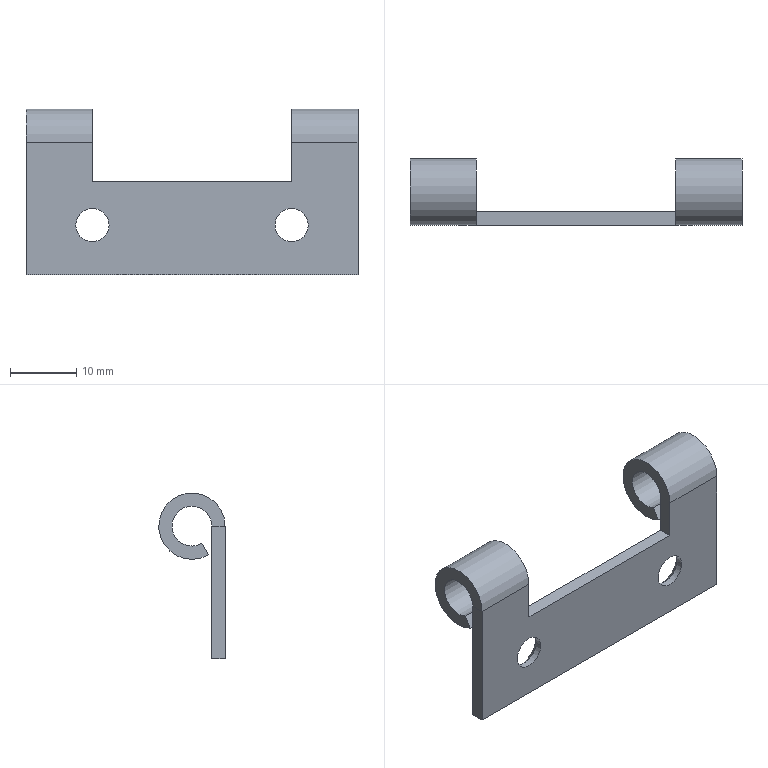Component | SolidWorks | Hinge-1_Hinge1-1 | 1 solid | 24 faces | box 50 x 10 x 25 mm | volume 2381 mm3 | plane 12 | cylinder 8 | cone 4 | commonest cylinder face diameters 5 x4 6 x2 10 x2
STEP:
#1=CARTESIAN_POINT('',(47.547,58.634,57.439));
#2=VERTEX_POINT('',#1);
#3=CARTESIAN_POINT('',(47.35,58.634,57.439));
#4=VERTEX_POINT('',#3);
#5=CARTESIAN_POINT('',(47.448,58.634,57.439));
#6=DIRECTION('',(0.,1.,0.));
#7=DIRECTION('',(-1.,0.,0.));
#8=AXIS2_PLACEMENT_3D('',#5,#6,#7);
#9=CIRCLE('',#8,0.09843);
#10=EDGE_CURVE('',#2,#4,#9,.T.);
#11=ORIENTED_EDGE('',*,*,#10,.F.);
#12=CARTESIAN_POINT('',(47.586,58.674,57.439));
#13=VERTEX_POINT('',#12);
#14=CARTESIAN_POINT('',(47.586,58.674,57.439));
#15=DIRECTION('',(0.7071,0.7071,0.));
#16=VECTOR('',#15,39.37);
#17=LINE('',#14,#16);
#18=EDGE_CURVE('',#2,#13,#17,.T.);
#19=ORIENTED_EDGE('',*,*,#18,.T.);
#20=CARTESIAN_POINT('',(47.31,58.674,57.439));
#21=VERTEX_POINT('',#20);
#22=CARTESIAN_POINT('',(47.448,58.674,57.439));
#23=DIRECTION('',(0.,-1.,-0.));
#24=DIRECTION('',(-1.,0.,0.));
#25=AXIS2_PLACEMENT_3D('',#22,#23,#24);
#26=CIRCLE('',#25,0.1378);
#27=EDGE_CURVE('',#21,#13,#26,.T.);
#28=ORIENTED_EDGE('',*,*,#27,.F.);
#29=CARTESIAN_POINT('',(47.31,58.674,57.439));
#30=DIRECTION('',(-0.7071,0.7071,0.));
#31=VECTOR('',#30,39.37);
#32=LINE('',#29,#31);
#33=EDGE_CURVE('',#4,#21,#32,.T.);
#34=ORIENTED_EDGE('',*,*,#33,.F.);
#35=EDGE_LOOP('',(#11,#19,#28,#34));
#36=FACE_OUTER_BOUND('',#35,.T.);
#37=CARTESIAN_POINT('',(47.448,58.674,57.439));
#38=DIRECTION('',(0.,1.,0.));
#39=DIRECTION('',(-1.,0.,0.));
#40=AXIS2_PLACEMENT_3D('',#37,#38,#39);
#41=CONICAL_SURFACE('',#40,0.1378,0.7854);
#42=ADVANCED_FACE('',(#36),#41,.F.);
#43=CARTESIAN_POINT('',(46.366,58.634,57.439));
#44=VERTEX_POINT('',#43);
#45=CARTESIAN_POINT('',(46.169,58.634,57.439));
#46=VERTEX_POINT('',#45);
#47=CARTESIAN_POINT('',(46.267,58.634,57.439));
#48=DIRECTION('',(0.,1.,0.));
#49=DIRECTION('',(-1.,0.,0.));
#50=AXIS2_PLACEMENT_3D('',#47,#48,#49);
#51=CIRCLE('',#50,0.09843);
#52=EDGE_CURVE('',#44,#46,#51,.T.);
#53=ORIENTED_EDGE('',*,*,#52,.F.);
#54=CARTESIAN_POINT('',(46.405,58.674,57.439));
#55=VERTEX_POINT('',#54);
#56=CARTESIAN_POINT('',(46.405,58.674,57.439));
#57=DIRECTION('',(0.7071,0.7071,0.));
#58=VECTOR('',#57,39.37);
#59=LINE('',#56,#58);
#60=EDGE_CURVE('',#44,#55,#59,.T.);
#61=ORIENTED_EDGE('',*,*,#60,.T.);
#62=CARTESIAN_POINT('',(46.129,58.674,57.439));
#63=VERTEX_POINT('',#62);
#64=CARTESIAN_POINT('',(46.267,58.674,57.439));
#65=DIRECTION('',(0.,-1.,-0.));
#66=DIRECTION('',(-1.,0.,0.));
#67=AXIS2_PLACEMENT_3D('',#64,#65,#66);
#68=CIRCLE('',#67,0.1378);
#69=EDGE_CURVE('',#63,#55,#68,.T.);
#70=ORIENTED_EDGE('',*,*,#69,.F.);
#71=CARTESIAN_POINT('',(46.129,58.674,57.439));
#72=DIRECTION('',(-0.7071,0.7071,0.));
#73=VECTOR('',#72,39.37);
#74=LINE('',#71,#73);
#75=EDGE_CURVE('',#46,#63,#74,.T.);
#76=ORIENTED_EDGE('',*,*,#75,.F.);
#77=EDGE_LOOP('',(#53,#61,#70,#76));
#78=FACE_OUTER_BOUND('',#77,.T.);
#79=CARTESIAN_POINT('',(46.267,58.674,57.439));
#80=DIRECTION('',(0.,1.,0.));
#81=DIRECTION('',(-1.,0.,0.));
#82=AXIS2_PLACEMENT_3D('',#79,#80,#81);
#83=CONICAL_SURFACE('',#82,0.1378,0.7854);
#84=ADVANCED_FACE('',(#78),#83,.F.);
#85=ORIENTED_EDGE('',*,*,#52,.T.);
#86=CARTESIAN_POINT('',(46.169,58.595,57.439));
#87=VERTEX_POINT('',#86);
#88=CARTESIAN_POINT('',(46.169,58.989,57.439));
#89=DIRECTION('',(0.,-1.,-0.));
#90=VECTOR('',#89,39.37);
#91=LINE('',#88,#90);
#92=EDGE_CURVE('',#46,#87,#91,.T.);
#93=ORIENTED_EDGE('',*,*,#92,.T.);
#94=CARTESIAN_POINT('',(46.366,58.595,57.439));
#95=VERTEX_POINT('',#94);
#96=CARTESIAN_POINT('',(46.267,58.595,57.439));
#97=DIRECTION('',(0.,-1.,-0.));
#98=DIRECTION('',(1.,0.,0.));
#99=AXIS2_PLACEMENT_3D('',#96,#97,#98);
#100=CIRCLE('',#99,0.09843);
#101=EDGE_CURVE('',#87,#95,#100,.T.);
#102=ORIENTED_EDGE('',*,*,#101,.T.);
#103=CARTESIAN_POINT('',(46.366,58.989,57.439));
#104=DIRECTION('',(0.,-1.,-0.));
#105=VECTOR('',#104,39.37);
#106=LINE('',#103,#105);
#107=EDGE_CURVE('',#44,#95,#106,.T.);
#108=ORIENTED_EDGE('',*,*,#107,.F.);
#109=EDGE_LOOP('',(#85,#93,#102,#108));
#110=FACE_OUTER_BOUND('',#109,.T.);
#111=CARTESIAN_POINT('',(46.267,58.989,57.439));
#112=DIRECTION('',(0.,-1.,-0.));
#113=DIRECTION('',(1.,0.,0.));
#114=AXIS2_PLACEMENT_3D('',#111,#112,#113);
#115=CYLINDRICAL_SURFACE('',#114,0.09843);
#116=ADVANCED_FACE('',(#110),#115,.F.);
#117=ORIENTED_EDGE('',*,*,#10,.T.);
#118=CARTESIAN_POINT('',(47.35,58.595,57.439));
#119=VERTEX_POINT('',#118);
#120=CARTESIAN_POINT('',(47.35,58.989,57.439));
#121=DIRECTION('',(0.,-1.,-0.));
#122=VECTOR('',#121,39.37);
#123=LINE('',#120,#122);
#124=EDGE_CURVE('',#4,#119,#123,.T.);
#125=ORIENTED_EDGE('',*,*,#124,.T.);
#126=CARTESIAN_POINT('',(47.547,58.595,57.439));
#127=VERTEX_POINT('',#126);
#128=CARTESIAN_POINT('',(47.448,58.595,57.439));
#129=DIRECTION('',(0.,-1.,-0.));
#130=DIRECTION('',(1.,0.,0.));
#131=AXIS2_PLACEMENT_3D('',#128,#129,#130);
#132=CIRCLE('',#131,0.09843);
#133=EDGE_CURVE('',#119,#127,#132,.T.);
#134=ORIENTED_EDGE('',*,*,#133,.T.);
#135=CARTESIAN_POINT('',(47.547,58.989,57.439));
#136=DIRECTION('',(0.,-1.,-0.));
#137=VECTOR('',#136,39.37);
#138=LINE('',#135,#137);
#139=EDGE_CURVE('',#2,#127,#138,.T.);
#140=ORIENTED_EDGE('',*,*,#139,.F.);
#141=EDGE_LOOP('',(#117,#125,#134,#140));
#142=FACE_OUTER_BOUND('',#141,.T.);
#143=CARTESIAN_POINT('',(47.448,58.989,57.439));
#144=DIRECTION('',(0.,-1.,-0.));
#145=DIRECTION('',(1.,0.,0.));
#146=AXIS2_PLACEMENT_3D('',#143,#144,#145);
#147=CYLINDRICAL_SURFACE('',#146,0.09843);
#148=ADVANCED_FACE('',(#142),#147,.F.);
#149=CARTESIAN_POINT('',(47.448,58.733,57.829));
#150=VERTEX_POINT('',#149);
#151=CARTESIAN_POINT('',(47.448,58.674,57.931));
#152=VERTEX_POINT('',#151);
#153=CARTESIAN_POINT('',(47.448,58.792,57.931));
#154=DIRECTION('',(1.,0.,0.));
#155=DIRECTION('',(0.,1.,0.));
#156=AXIS2_PLACEMENT_3D('',#153,#154,#155);
#157=CIRCLE('',#156,0.1181);
#158=EDGE_CURVE('',#150,#152,#157,.T.);
#159=ORIENTED_EDGE('',*,*,#158,.F.);
#160=CARTESIAN_POINT('',(47.842,58.733,57.829));
#161=VERTEX_POINT('',#160);
#162=CARTESIAN_POINT('',(47.842,58.733,57.829));
#163=DIRECTION('',(-1.,0.,0.));
#164=VECTOR('',#163,39.37);
#165=LINE('',#162,#164);
#166=EDGE_CURVE('',#161,#150,#165,.T.);
#167=ORIENTED_EDGE('',*,*,#166,.F.);
#168=CARTESIAN_POINT('',(47.842,58.674,57.931));
#169=VERTEX_POINT('',#168);
#170=CARTESIAN_POINT('',(47.842,58.792,57.931));
#171=DIRECTION('',(1.,0.,0.));
#172=DIRECTION('',(0.,1.,0.));
#173=AXIS2_PLACEMENT_3D('',#170,#171,#172);
#174=CIRCLE('',#173,0.1181);
#175=EDGE_CURVE('',#161,#169,#174,.T.);
#176=ORIENTED_EDGE('',*,*,#175,.T.);
#177=CARTESIAN_POINT('',(47.842,58.674,57.931));
#178=DIRECTION('',(-1.,0.,0.));
#179=VECTOR('',#178,39.37);
#180=LINE('',#177,#179);
#181=EDGE_CURVE('',#169,#152,#180,.T.);
#182=ORIENTED_EDGE('',*,*,#181,.T.);
#183=EDGE_LOOP('',(#159,#167,#176,#182));
#184=FACE_OUTER_BOUND('',#183,.T.);
#185=CARTESIAN_POINT('',(47.842,58.792,57.931));
#186=DIRECTION('',(-1.,0.,0.));
#187=DIRECTION('',(0.,-1.,0.));
#188=AXIS2_PLACEMENT_3D('',#185,#186,#187);
#189=CYLINDRICAL_SURFACE('',#188,0.1181);
#190=ADVANCED_FACE('',(#184),#189,.F.);
#191=CARTESIAN_POINT('',(47.448,58.693,57.761));
#192=VERTEX_POINT('',#191);
#193=CARTESIAN_POINT('',(47.448,58.693,57.761));
#194=DIRECTION('',(0.,0.5,0.866));
#195=VECTOR('',#194,39.37);
#196=LINE('',#193,#195);
#197=EDGE_CURVE('',#192,#150,#196,.T.);
#198=ORIENTED_EDGE('',*,*,#197,.F.);
#199=CARTESIAN_POINT('',(47.842,58.693,57.761));
#200=VERTEX_POINT('',#199);
#201=CARTESIAN_POINT('',(47.842,58.693,57.761));
#202=DIRECTION('',(-1.,0.,0.));
#203=VECTOR('',#202,39.37);
#204=LINE('',#201,#203);
#205=EDGE_CURVE('',#200,#192,#204,.T.);
#206=ORIENTED_EDGE('',*,*,#205,.F.);
#207=CARTESIAN_POINT('',(47.842,58.693,57.761));
#208=DIRECTION('',(0.,0.5,0.866));
#209=VECTOR('',#208,39.37);
#210=LINE('',#207,#209);
#211=EDGE_CURVE('',#200,#161,#210,.T.);
#212=ORIENTED_EDGE('',*,*,#211,.T.);
#213=ORIENTED_EDGE('',*,*,#166,.T.);
#214=EDGE_LOOP('',(#198,#206,#212,#213));
#215=FACE_OUTER_BOUND('',#214,.T.);
#216=CARTESIAN_POINT('',(47.842,58.693,57.761));
#217=DIRECTION('',(0.,-0.866,0.5));
#218=DIRECTION('',(0.,-0.5,-0.866));
#219=AXIS2_PLACEMENT_3D('',#216,#217,#218);
#220=PLANE('',#219);
#221=ADVANCED_FACE('',(#215),#220,.T.);
#222=CARTESIAN_POINT('',(47.448,58.595,57.931));
#223=VERTEX_POINT('',#222);
#224=CARTESIAN_POINT('',(47.448,58.792,57.931));
#225=DIRECTION('',(1.,0.,0.));
#226=DIRECTION('',(0.,1.,0.));
#227=AXIS2_PLACEMENT_3D('',#224,#225,#226);
#228=CIRCLE('',#227,0.1969);
#229=EDGE_CURVE('',#192,#223,#228,.T.);
#230=ORIENTED_EDGE('',*,*,#229,.T.);
#231=CARTESIAN_POINT('',(47.842,58.595,57.931));
#232=VERTEX_POINT('',#231);
#233=CARTESIAN_POINT('',(47.842,58.595,57.931));
#234=DIRECTION('',(-1.,0.,0.));
#235=VECTOR('',#234,39.37);
#236=LINE('',#233,#235);
#237=EDGE_CURVE('',#232,#223,#236,.T.);
#238=ORIENTED_EDGE('',*,*,#237,.F.);
#239=CARTESIAN_POINT('',(47.842,58.792,57.931));
#240=DIRECTION('',(1.,0.,0.));
#241=DIRECTION('',(0.,1.,0.));
#242=AXIS2_PLACEMENT_3D('',#239,#240,#241);
#243=CIRCLE('',#242,0.1969);
#244=EDGE_CURVE('',#200,#232,#243,.T.);
#245=ORIENTED_EDGE('',*,*,#244,.F.);
#246=ORIENTED_EDGE('',*,*,#205,.T.);
#247=EDGE_LOOP('',(#230,#238,#245,#246));
#248=FACE_OUTER_BOUND('',#247,.T.);
#249=CARTESIAN_POINT('',(47.842,58.792,57.931));
#250=DIRECTION('',(-1.,0.,0.));
#251=DIRECTION('',(0.,-1.,0.));
#252=AXIS2_PLACEMENT_3D('',#249,#250,#251);
#253=CYLINDRICAL_SURFACE('',#252,0.1969);
#254=ADVANCED_FACE('',(#248),#253,.T.);
#255=CARTESIAN_POINT('',(47.842,58.674,57.931));
#256=DIRECTION('',(0.,-1.,-0.));
#257=VECTOR('',#256,39.37);
#258=LINE('',#255,#257);
#259=EDGE_CURVE('',#169,#232,#258,.T.);
#260=ORIENTED_EDGE('',*,*,#259,.F.);
#261=ORIENTED_EDGE('',*,*,#175,.F.);
#262=ORIENTED_EDGE('',*,*,#211,.F.);
#263=ORIENTED_EDGE('',*,*,#244,.T.);
#264=EDGE_LOOP('',(#260,#261,#262,#263));
#265=FACE_OUTER_BOUND('',#264,.T.);
#266=CARTESIAN_POINT('',(47.842,58.674,57.931));
#267=DIRECTION('',(1.,0.,0.));
#268=DIRECTION('',(0.,1.,0.));
#269=AXIS2_PLACEMENT_3D('',#266,#267,#268);
#270=PLANE('',#269);
#271=ADVANCED_FACE('',(#265),#270,.T.);
#272=CARTESIAN_POINT('',(45.873,58.595,57.931));
#273=VERTEX_POINT('',#272);
#274=CARTESIAN_POINT('',(45.873,58.674,57.931));
#275=VERTEX_POINT('',#274);
#276=CARTESIAN_POINT('',(45.873,58.595,57.931));
#277=DIRECTION('',(0.,1.,0.));
#278=VECTOR('',#277,39.37);
#279=LINE('',#276,#278);
#280=EDGE_CURVE('',#273,#275,#279,.T.);
#281=ORIENTED_EDGE('',*,*,#280,.F.);
#282=CARTESIAN_POINT('',(45.873,58.693,57.761));
#283=VERTEX_POINT('',#282);
#284=CARTESIAN_POINT('',(45.873,58.792,57.931));
#285=DIRECTION('',(1.,0.,0.));
#286=DIRECTION('',(0.,1.,0.));
#287=AXIS2_PLACEMENT_3D('',#284,#285,#286);
#288=CIRCLE('',#287,0.1969);
#289=EDGE_CURVE('',#283,#273,#288,.T.);
#290=ORIENTED_EDGE('',*,*,#289,.F.);
#291=CARTESIAN_POINT('',(45.873,58.733,57.829));
#292=VERTEX_POINT('',#291);
#293=CARTESIAN_POINT('',(45.873,58.693,57.761));
#294=DIRECTION('',(0.,0.5,0.866));
#295=VECTOR('',#294,39.37);
#296=LINE('',#293,#295);
#297=EDGE_CURVE('',#283,#292,#296,.T.);
#298=ORIENTED_EDGE('',*,*,#297,.T.);
#299=CARTESIAN_POINT('',(45.873,58.792,57.931));
#300=DIRECTION('',(1.,0.,0.));
#301=DIRECTION('',(0.,1.,0.));
#302=AXIS2_PLACEMENT_3D('',#299,#300,#301);
#303=CIRCLE('',#302,0.1181);
#304=EDGE_CURVE('',#292,#275,#303,.T.);
#305=ORIENTED_EDGE('',*,*,#304,.T.);
#306=EDGE_LOOP('',(#281,#290,#298,#305));
#307=FACE_OUTER_BOUND('',#306,.T.);
#308=CARTESIAN_POINT('',(45.873,58.595,57.931));
#309=DIRECTION('',(-1.,0.,0.));
#310=DIRECTION('',(0.,-1.,-0.));
#311=AXIS2_PLACEMENT_3D('',#308,#309,#310);
#312=PLANE('',#311);
#313=ADVANCED_FACE('',(#307),#312,.T.);
#314=CARTESIAN_POINT('',(46.267,58.595,57.439));
#315=DIRECTION('',(0.,-1.,-0.));
#316=DIRECTION('',(1.,0.,0.));
#317=AXIS2_PLACEMENT_3D('',#314,#315,#316);
#318=CIRCLE('',#317,0.09843);
#319=EDGE_CURVE('',#95,#87,#318,.T.);
#320=ORIENTED_EDGE('',*,*,#319,.F.);
#321=ORIENTED_EDGE('',*,*,#101,.F.);
#322=EDGE_LOOP('',(#320,#321));
#323=FACE_BOUND('',#322,.T.);
#324=CARTESIAN_POINT('',(47.448,58.595,57.439));
#325=DIRECTION('',(0.,-1.,-0.));
#326=DIRECTION('',(1.,0.,0.));
#327=AXIS2_PLACEMENT_3D('',#324,#325,#326);
#328=CIRCLE('',#327,0.09843);
#329=EDGE_CURVE('',#127,#119,#328,.T.);
#330=ORIENTED_EDGE('',*,*,#329,.F.);
#331=ORIENTED_EDGE('',*,*,#133,.F.);
#332=EDGE_LOOP('',(#330,#331));
#333=FACE_BOUND('',#332,.T.);
#334=ORIENTED_EDGE('',*,*,#237,.T.);
#335=CARTESIAN_POINT('',(47.448,58.595,57.695));
#336=VERTEX_POINT('',#335);
#337=CARTESIAN_POINT('',(47.448,58.595,58.167));
#338=DIRECTION('',(0.,-0.,1.));
#339=VECTOR('',#338,39.37);
#340=LINE('',#337,#339);
#341=EDGE_CURVE('',#336,#223,#340,.T.);
#342=ORIENTED_EDGE('',*,*,#341,.F.);
#343=CARTESIAN_POINT('',(46.267,58.595,57.695));
#344=VERTEX_POINT('',#343);
#345=CARTESIAN_POINT('',(46.267,58.595,57.695));
#346=DIRECTION('',(1.,0.,0.));
#347=VECTOR('',#346,39.37);
#348=LINE('',#345,#347);
#349=EDGE_CURVE('',#344,#336,#348,.T.);
#350=ORIENTED_EDGE('',*,*,#349,.F.);
#351=CARTESIAN_POINT('',(46.267,58.595,57.931));
#352=VERTEX_POINT('',#351);
#353=CARTESIAN_POINT('',(46.267,58.595,58.167));
#354=DIRECTION('',(0.,0.,-1.));
#355=VECTOR('',#354,39.37);
#356=LINE('',#353,#355);
#357=EDGE_CURVE('',#352,#344,#356,.T.);
#358=ORIENTED_EDGE('',*,*,#357,.F.);
#359=CARTESIAN_POINT('',(47.842,58.595,57.931));
#360=DIRECTION('',(-1.,0.,0.));
#361=VECTOR('',#360,39.37);
#362=LINE('',#359,#361);
#363=EDGE_CURVE('',#352,#273,#362,.T.);
#364=ORIENTED_EDGE('',*,*,#363,.T.);
#365=CARTESIAN_POINT('',(45.873,58.595,57.144));
#366=VERTEX_POINT('',#365);
#367=CARTESIAN_POINT('',(45.873,58.595,57.144));
#368=DIRECTION('',(0.,0.,-1.));
#369=VECTOR('',#368,39.37);
#370=LINE('',#367,#369);
#371=EDGE_CURVE('',#273,#366,#370,.T.);
#372=ORIENTED_EDGE('',*,*,#371,.T.);
#373=CARTESIAN_POINT('',(47.842,58.595,57.144));
#374=VERTEX_POINT('',#373);
#375=CARTESIAN_POINT('',(47.842,58.595,57.144));
#376=DIRECTION('',(-1.,0.,0.));
#377=VECTOR('',#376,39.37);
#378=LINE('',#375,#377);
#379=EDGE_CURVE('',#374,#366,#378,.T.);
#380=ORIENTED_EDGE('',*,*,#379,.F.);
#381=CARTESIAN_POINT('',(47.842,58.595,57.144));
#382=DIRECTION('',(0.,0.,-1.));
#383=VECTOR('',#382,39.37);
#384=LINE('',#381,#383);
#385=EDGE_CURVE('',#232,#374,#384,.T.);
#386=ORIENTED_EDGE('',*,*,#385,.F.);
#387=EDGE_LOOP('',(#334,#342,#350,#358,#364,#372,#380,#386));
#388=FACE_OUTER_BOUND('',#387,.T.);
#389=CARTESIAN_POINT('',(47.842,58.595,57.144));
#390=DIRECTION('',(0.,1.,0.));
#391=DIRECTION('',(-1.,0.,0.));
#392=AXIS2_PLACEMENT_3D('',#389,#390,#391);
#393=PLANE('',#392);
#394=ADVANCED_FACE('',(#323,#333,#388),#393,.F.);
#395=CARTESIAN_POINT('',(45.873,58.674,57.144));
#396=VERTEX_POINT('',#395);
#397=CARTESIAN_POINT('',(45.873,58.674,57.144));
#398=DIRECTION('',(0.,-1.,-0.));
#399=VECTOR('',#398,39.37);
#400=LINE('',#397,#399);
#401=EDGE_CURVE('',#396,#366,#400,.T.);
#402=ORIENTED_EDGE('',*,*,#401,.F.);
#403=CARTESIAN_POINT('',(47.842,58.674,57.144));
#404=VERTEX_POINT('',#403);
#405=CARTESIAN_POINT('',(47.842,58.674,57.144));
#406=DIRECTION('',(-1.,0.,0.));
#407=VECTOR('',#406,39.37);
#408=LINE('',#405,#407);
#409=EDGE_CURVE('',#404,#396,#408,.T.);
#410=ORIENTED_EDGE('',*,*,#409,.F.);
#411=CARTESIAN_POINT('',(47.842,58.674,57.144));
#412=DIRECTION('',(0.,-1.,-0.));
#413=VECTOR('',#412,39.37);
#414=LINE('',#411,#413);
#415=EDGE_CURVE('',#404,#374,#414,.T.);
#416=ORIENTED_EDGE('',*,*,#415,.T.);
#417=ORIENTED_EDGE('',*,*,#379,.T.);
#418=EDGE_LOOP('',(#402,#410,#416,#417));
#419=FACE_OUTER_BOUND('',#418,.T.);
#420=CARTESIAN_POINT('',(47.842,58.674,57.144));
#421=DIRECTION('',(0.,0.,-1.));
#422=DIRECTION('',(0.,1.,0.));
#423=AXIS2_PLACEMENT_3D('',#420,#421,#422);
#424=PLANE('',#423);
#425=ADVANCED_FACE('',(#419),#424,.T.);
#426=ORIENTED_EDGE('',*,*,#69,.T.);
#427=CARTESIAN_POINT('',(46.267,58.674,57.439));
#428=DIRECTION('',(0.,-1.,-0.));
#429=DIRECTION('',(-1.,0.,0.));
#430=AXIS2_PLACEMENT_3D('',#427,#428,#429);
#431=CIRCLE('',#430,0.1378);
#432=EDGE_CURVE('',#55,#63,#431,.T.);
#433=ORIENTED_EDGE('',*,*,#432,.T.);
#434=EDGE_LOOP('',(#426,#433));
#435=FACE_BOUND('',#434,.T.);
#436=ORIENTED_EDGE('',*,*,#27,.T.);
#437=CARTESIAN_POINT('',(47.448,58.674,57.439));
#438=DIRECTION('',(0.,-1.,-0.));
#439=DIRECTION('',(-1.,0.,0.));
#440=AXIS2_PLACEMENT_3D('',#437,#438,#439);
#441=CIRCLE('',#440,0.1378);
#442=EDGE_CURVE('',#13,#21,#441,.T.);
#443=ORIENTED_EDGE('',*,*,#442,.T.);
#444=EDGE_LOOP('',(#436,#443));
#445=FACE_BOUND('',#444,.T.);
#446=CARTESIAN_POINT('',(47.448,58.674,57.695));
#447=VERTEX_POINT('',#446);
#448=CARTESIAN_POINT('',(47.448,58.674,57.144));
#449=DIRECTION('',(0.,0.,-1.));
#450=VECTOR('',#449,39.37);
#451=LINE('',#448,#450);
#452=EDGE_CURVE('',#152,#447,#451,.T.);
#453=ORIENTED_EDGE('',*,*,#452,.F.);
#454=ORIENTED_EDGE('',*,*,#181,.F.);
#455=CARTESIAN_POINT('',(47.842,58.674,57.144));
#456=DIRECTION('',(0.,0.,-1.));
#457=VECTOR('',#456,39.37);
#458=LINE('',#455,#457);
#459=EDGE_CURVE('',#169,#404,#458,.T.);
#460=ORIENTED_EDGE('',*,*,#459,.T.);
#461=ORIENTED_EDGE('',*,*,#409,.T.);
#462=CARTESIAN_POINT('',(45.873,58.674,57.144));
#463=DIRECTION('',(0.,0.,-1.));
#464=VECTOR('',#463,39.37);
#465=LINE('',#462,#464);
#466=EDGE_CURVE('',#275,#396,#465,.T.);
#467=ORIENTED_EDGE('',*,*,#466,.F.);
#468=CARTESIAN_POINT('',(46.267,58.674,57.931));
#469=VERTEX_POINT('',#468);
#470=CARTESIAN_POINT('',(47.842,58.674,57.931));
#471=DIRECTION('',(-1.,0.,0.));
#472=VECTOR('',#471,39.37);
#473=LINE('',#470,#472);
#474=EDGE_CURVE('',#469,#275,#473,.T.);
#475=ORIENTED_EDGE('',*,*,#474,.F.);
#476=CARTESIAN_POINT('',(46.267,58.674,57.695));
#477=VERTEX_POINT('',#476);
#478=CARTESIAN_POINT('',(46.267,58.674,57.144));
#479=DIRECTION('',(0.,-0.,1.));
#480=VECTOR('',#479,39.37);
#481=LINE('',#478,#480);
#482=EDGE_CURVE('',#477,#469,#481,.T.);
#483=ORIENTED_EDGE('',*,*,#482,.F.);
#484=CARTESIAN_POINT('',(47.842,58.674,57.695));
#485=DIRECTION('',(-1.,0.,0.));
#486=VECTOR('',#485,39.37);
#487=LINE('',#484,#486);
#488=EDGE_CURVE('',#447,#477,#487,.T.);
#489=ORIENTED_EDGE('',*,*,#488,.F.);
#490=EDGE_LOOP('',(#453,#454,#460,#461,#467,#475,#483,#489));
#491=FACE_OUTER_BOUND('',#490,.T.);
#492=CARTESIAN_POINT('',(47.842,58.674,57.144));
#493=DIRECTION('',(0.,1.,0.));
#494=DIRECTION('',(-1.,0.,0.));
#495=AXIS2_PLACEMENT_3D('',#492,#493,#494);
#496=PLANE('',#495);
#497=ADVANCED_FACE('',(#435,#445,#491),#496,.T.);
#498=CARTESIAN_POINT('',(46.267,58.733,57.829));
#499=VERTEX_POINT('',#498);
#500=CARTESIAN_POINT('',(46.267,58.792,57.931));
#501=DIRECTION('',(-1.,0.,0.));
#502=DIRECTION('',(0.,-1.,0.));
#503=AXIS2_PLACEMENT_3D('',#500,#501,#502);
#504=CIRCLE('',#503,0.1181);
#505=EDGE_CURVE('',#469,#499,#504,.T.);
#506=ORIENTED_EDGE('',*,*,#505,.F.);
#507=ORIENTED_EDGE('',*,*,#474,.T.);
#508=ORIENTED_EDGE('',*,*,#304,.F.);
#509=CARTESIAN_POINT('',(47.842,58.733,57.829));
#510=DIRECTION('',(-1.,0.,0.));
#511=VECTOR('',#510,39.37);
#512=LINE('',#509,#511);
#513=EDGE_CURVE('',#499,#292,#512,.T.);
#514=ORIENTED_EDGE('',*,*,#513,.F.);
#515=EDGE_LOOP('',(#506,#507,#508,#514));
#516=FACE_OUTER_BOUND('',#515,.T.);
#517=CARTESIAN_POINT('',(47.842,58.792,57.931));
#518=DIRECTION('',(-1.,0.,0.));
#519=DIRECTION('',(0.,-1.,0.));
#520=AXIS2_PLACEMENT_3D('',#517,#518,#519);
#521=CYLINDRICAL_SURFACE('',#520,0.1181);
#522=ADVANCED_FACE('',(#516),#521,.F.);
#523=CARTESIAN_POINT('',(46.267,58.693,57.761));
#524=VERTEX_POINT('',#523);
#525=CARTESIAN_POINT('',(46.267,58.693,57.761));
#526=DIRECTION('',(0.,-0.5,-0.866));
#527=VECTOR('',#526,39.37);
#528=LINE('',#525,#527);
#529=EDGE_CURVE('',#499,#524,#528,.T.);
#530=ORIENTED_EDGE('',*,*,#529,.F.);
#531=ORIENTED_EDGE('',*,*,#513,.T.);
#532=ORIENTED_EDGE('',*,*,#297,.F.);
#533=CARTESIAN_POINT('',(47.842,58.693,57.761));
#534=DIRECTION('',(-1.,0.,0.));
#535=VECTOR('',#534,39.37);
#536=LINE('',#533,#535);
#537=EDGE_CURVE('',#524,#283,#536,.T.);
#538=ORIENTED_EDGE('',*,*,#537,.F.);
#539=EDGE_LOOP('',(#530,#531,#532,#538));
#540=FACE_OUTER_BOUND('',#539,.T.);
#541=CARTESIAN_POINT('',(47.842,58.693,57.761));
#542=DIRECTION('',(0.,-0.866,0.5));
#543=DIRECTION('',(0.,-0.5,-0.866));
#544=AXIS2_PLACEMENT_3D('',#541,#542,#543);
#545=PLANE('',#544);
#546=ADVANCED_FACE('',(#540),#545,.T.);
#547=ORIENTED_EDGE('',*,*,#363,.F.);
#548=CARTESIAN_POINT('',(46.267,58.792,57.931));
#549=DIRECTION('',(-1.,0.,0.));
#550=DIRECTION('',(0.,-1.,0.));
#551=AXIS2_PLACEMENT_3D('',#548,#549,#550);
#552=CIRCLE('',#551,0.1969);
#553=EDGE_CURVE('',#352,#524,#552,.T.);
#554=ORIENTED_EDGE('',*,*,#553,.T.);
#555=ORIENTED_EDGE('',*,*,#537,.T.);
#556=ORIENTED_EDGE('',*,*,#289,.T.);
#557=EDGE_LOOP('',(#547,#554,#555,#556));
#558=FACE_OUTER_BOUND('',#557,.T.);
#559=CARTESIAN_POINT('',(47.842,58.792,57.931));
#560=DIRECTION('',(-1.,0.,0.));
#561=DIRECTION('',(0.,-1.,0.));
#562=AXIS2_PLACEMENT_3D('',#559,#560,#561);
#563=CYLINDRICAL_SURFACE('',#562,0.1969);
#564=ADVANCED_FACE('',(#558),#563,.T.);
#565=ORIENTED_EDGE('',*,*,#385,.T.);
#566=ORIENTED_EDGE('',*,*,#415,.F.);
#567=ORIENTED_EDGE('',*,*,#459,.F.);
#568=ORIENTED_EDGE('',*,*,#259,.T.);
#569=EDGE_LOOP('',(#565,#566,#567,#568));
#570=FACE_OUTER_BOUND('',#569,.T.);
#571=CARTESIAN_POINT('',(47.842,58.792,57.931));
#572=DIRECTION('',(1.,0.,0.));
#573=DIRECTION('',(0.,1.,0.));
#574=AXIS2_PLACEMENT_3D('',#571,#572,#573);
#575=PLANE('',#574);
#576=ADVANCED_FACE('',(#570),#575,.T.);
#577=ORIENTED_EDGE('',*,*,#371,.F.);
#578=ORIENTED_EDGE('',*,*,#280,.T.);
#579=ORIENTED_EDGE('',*,*,#466,.T.);
#580=ORIENTED_EDGE('',*,*,#401,.T.);
#581=EDGE_LOOP('',(#577,#578,#579,#580));
#582=FACE_OUTER_BOUND('',#581,.T.);
#583=CARTESIAN_POINT('',(45.873,58.792,57.931));
#584=DIRECTION('',(1.,0.,0.));
#585=DIRECTION('',(0.,1.,0.));
#586=AXIS2_PLACEMENT_3D('',#583,#584,#585);
#587=PLANE('',#586);
#588=ADVANCED_FACE('',(#582),#587,.F.);
#589=ORIENTED_EDGE('',*,*,#452,.T.);
#590=CARTESIAN_POINT('',(47.448,58.989,57.695));
#591=DIRECTION('',(0.,-1.,-0.));
#592=VECTOR('',#591,39.37);
#593=LINE('',#590,#592);
#594=EDGE_CURVE('',#447,#336,#593,.T.);
#595=ORIENTED_EDGE('',*,*,#594,.T.);
#596=ORIENTED_EDGE('',*,*,#341,.T.);
#597=ORIENTED_EDGE('',*,*,#229,.F.);
#598=ORIENTED_EDGE('',*,*,#197,.T.);
#599=ORIENTED_EDGE('',*,*,#158,.T.);
#600=EDGE_LOOP('',(#589,#595,#596,#597,#598,#599));
#601=FACE_OUTER_BOUND('',#600,.T.);
#602=CARTESIAN_POINT('',(47.448,58.989,58.167));
#603=DIRECTION('',(1.,0.,0.));
#604=DIRECTION('',(0.,1.,0.));
#605=AXIS2_PLACEMENT_3D('',#602,#603,#604);
#606=PLANE('',#605);
#607=ADVANCED_FACE('',(#601),#606,.F.);
#608=ORIENTED_EDGE('',*,*,#482,.T.);
#609=ORIENTED_EDGE('',*,*,#505,.T.);
#610=ORIENTED_EDGE('',*,*,#529,.T.);
#611=ORIENTED_EDGE('',*,*,#553,.F.);
#612=ORIENTED_EDGE('',*,*,#357,.T.);
#613=CARTESIAN_POINT('',(46.267,58.989,57.695));
#614=DIRECTION('',(0.,-1.,-0.));
#615=VECTOR('',#614,39.37);
#616=LINE('',#613,#615);
#617=EDGE_CURVE('',#477,#344,#616,.T.);
#618=ORIENTED_EDGE('',*,*,#617,.F.);
#619=EDGE_LOOP('',(#608,#609,#610,#611,#612,#618));
#620=FACE_OUTER_BOUND('',#619,.T.);
#621=CARTESIAN_POINT('',(46.267,58.989,58.167));
#622=DIRECTION('',(-1.,0.,0.));
#623=DIRECTION('',(0.,-1.,-0.));
#624=AXIS2_PLACEMENT_3D('',#621,#622,#623);
#625=PLANE('',#624);
#626=ADVANCED_FACE('',(#620),#625,.F.);
#627=ORIENTED_EDGE('',*,*,#488,.T.);
#628=ORIENTED_EDGE('',*,*,#617,.T.);
#629=ORIENTED_EDGE('',*,*,#349,.T.);
#630=ORIENTED_EDGE('',*,*,#594,.F.);
#631=EDGE_LOOP('',(#627,#628,#629,#630));
#632=FACE_OUTER_BOUND('',#631,.T.);
#633=CARTESIAN_POINT('',(46.267,58.989,57.695));
#634=DIRECTION('',(0.,0.,-1.));
#635=DIRECTION('',(0.,1.,0.));
#636=AXIS2_PLACEMENT_3D('',#633,#634,#635);
#637=PLANE('',#636);
#638=ADVANCED_FACE('',(#632),#637,.F.);
#639=ORIENTED_EDGE('',*,*,#124,.F.);
#640=CARTESIAN_POINT('',(47.448,58.634,57.439));
#641=DIRECTION('',(0.,1.,0.));
#642=DIRECTION('',(-1.,0.,0.));
#643=AXIS2_PLACEMENT_3D('',#640,#641,#642);
#644=CIRCLE('',#643,0.09843);
#645=EDGE_CURVE('',#4,#2,#644,.T.);
#646=ORIENTED_EDGE('',*,*,#645,.T.);
#647=ORIENTED_EDGE('',*,*,#139,.T.);
#648=ORIENTED_EDGE('',*,*,#329,.T.);
#649=EDGE_LOOP('',(#639,#646,#647,#648));
#650=FACE_OUTER_BOUND('',#649,.T.);
#651=CARTESIAN_POINT('',(47.448,58.989,57.439));
#652=DIRECTION('',(0.,-1.,-0.));
#653=DIRECTION('',(1.,0.,0.));
#654=AXIS2_PLACEMENT_3D('',#651,#652,#653);
#655=CYLINDRICAL_SURFACE('',#654,0.09843);
#656=ADVANCED_FACE('',(#650),#655,.F.);
#657=ORIENTED_EDGE('',*,*,#92,.F.);
#658=CARTESIAN_POINT('',(46.267,58.634,57.439));
#659=DIRECTION('',(0.,1.,0.));
#660=DIRECTION('',(-1.,0.,0.));
#661=AXIS2_PLACEMENT_3D('',#658,#659,#660);
#662=CIRCLE('',#661,0.09843);
#663=EDGE_CURVE('',#46,#44,#662,.T.);
#664=ORIENTED_EDGE('',*,*,#663,.T.);
#665=ORIENTED_EDGE('',*,*,#107,.T.);
#666=ORIENTED_EDGE('',*,*,#319,.T.);
#667=EDGE_LOOP('',(#657,#664,#665,#666));
#668=FACE_OUTER_BOUND('',#667,.T.);
#669=CARTESIAN_POINT('',(46.267,58.989,57.439));
#670=DIRECTION('',(0.,-1.,-0.));
#671=DIRECTION('',(1.,0.,0.));
#672=AXIS2_PLACEMENT_3D('',#669,#670,#671);
#673=CYLINDRICAL_SURFACE('',#672,0.09843);
#674=ADVANCED_FACE('',(#668),#673,.F.);
#675=ORIENTED_EDGE('',*,*,#60,.F.);
#676=ORIENTED_EDGE('',*,*,#663,.F.);
#677=ORIENTED_EDGE('',*,*,#75,.T.);
#678=ORIENTED_EDGE('',*,*,#432,.F.);
#679=EDGE_LOOP('',(#675,#676,#677,#678));
#680=FACE_OUTER_BOUND('',#679,.T.);
#681=CARTESIAN_POINT('',(46.267,58.674,57.439));
#682=DIRECTION('',(0.,1.,0.));
#683=DIRECTION('',(-1.,0.,0.));
#684=AXIS2_PLACEMENT_3D('',#681,#682,#683);
#685=CONICAL_SURFACE('',#684,0.1378,0.7854);
#686=ADVANCED_FACE('',(#680),#685,.F.);
#687=ORIENTED_EDGE('',*,*,#18,.F.);
#688=ORIENTED_EDGE('',*,*,#645,.F.);
#689=ORIENTED_EDGE('',*,*,#33,.T.);
#690=ORIENTED_EDGE('',*,*,#442,.F.);
#691=EDGE_LOOP('',(#687,#688,#689,#690));
#692=FACE_OUTER_BOUND('',#691,.T.);
#693=CARTESIAN_POINT('',(47.448,58.674,57.439));
#694=DIRECTION('',(0.,1.,0.));
#695=DIRECTION('',(-1.,0.,0.));
#696=AXIS2_PLACEMENT_3D('',#693,#694,#695);
#697=CONICAL_SURFACE('',#696,0.1378,0.7854);
#698=ADVANCED_FACE('',(#692),#697,.F.);
#699=CLOSED_SHELL('',(#42,#84,#116,#148,#190,#221,#254,#271,#313,#394,#425,#497,#522,#546,#564,#576,#588,#607,#626,#638,#656,#674,#686,#698));
#700=MANIFOLD_SOLID_BREP('',#699);
#701=CARTESIAN_POINT('',(0.,0.,0.));
#702=DIRECTION('',(0.,0.,1.));
#703=DIRECTION('',(1.,0.,0.));
#704=AXIS2_PLACEMENT_3D('',#701,#702,#703);
#705=(LENGTH_UNIT()NAMED_UNIT(*)SI_UNIT($,.METRE.));
#706=LENGTH_MEASURE_WITH_UNIT(LENGTH_MEASURE(0.0254),#705);
#707=DIMENSIONAL_EXPONENTS(1.,0.,0.,0.,0.,0.,0.);
#708=(CONVERSION_BASED_UNIT('',#706)LENGTH_UNIT()NAMED_UNIT(#707));
#709=UNCERTAINTY_MEASURE_WITH_UNIT(LENGTH_MEASURE(0.00001),#708,'','');
#710=(NAMED_UNIT(*)PLANE_ANGLE_UNIT()SI_UNIT($,.RADIAN.));
#711=(NAMED_UNIT(*)SI_UNIT($,.STERADIAN.)SOLID_ANGLE_UNIT());
#712=(GEOMETRIC_REPRESENTATION_CONTEXT(3)GLOBAL_UNCERTAINTY_ASSIGNED_CONTEXT((#709))GLOBAL_UNIT_ASSIGNED_CONTEXT((#708,#710,#711))REPRESENTATION_CONTEXT('',''));
#713=ADVANCED_BREP_SHAPE_REPRESENTATION('',(#700,#704),#712);
#714=COLOUR_RGB('',0.7922,0.8196,0.9333);
#715=FILL_AREA_STYLE_COLOUR('',#714);
#716=FILL_AREA_STYLE('',(#715));
#717=SURFACE_STYLE_FILL_AREA(#716);
#718=SURFACE_SIDE_STYLE('',(#717));
#719=SURFACE_STYLE_USAGE(.BOTH.,#718);
#720=PRESENTATION_STYLE_ASSIGNMENT((#719));
#721=STYLED_ITEM('',(#720),#700);
#722=(LENGTH_UNIT()NAMED_UNIT(*)SI_UNIT($,.METRE.));
#723=LENGTH_MEASURE_WITH_UNIT(LENGTH_MEASURE(0.0254),#722);
#724=DIMENSIONAL_EXPONENTS(1.,0.,0.,0.,0.,0.,0.);
#725=(CONVERSION_BASED_UNIT('',#723)LENGTH_UNIT()NAMED_UNIT(#724));
#726=UNCERTAINTY_MEASURE_WITH_UNIT(LENGTH_MEASURE(0.00001),#725,'','');
#727=(NAMED_UNIT(*)PLANE_ANGLE_UNIT()SI_UNIT($,.RADIAN.));
#728=(NAMED_UNIT(*)SI_UNIT($,.STERADIAN.)SOLID_ANGLE_UNIT());
#729=(GEOMETRIC_REPRESENTATION_CONTEXT(3)GLOBAL_UNCERTAINTY_ASSIGNED_CONTEXT((#726))GLOBAL_UNIT_ASSIGNED_CONTEXT((#725,#727,#728))REPRESENTATION_CONTEXT('',''));
#730=MECHANICAL_DESIGN_GEOMETRIC_PRESENTATION_REPRESENTATION('',(#721),#729);
#731=PRESENTATION_LAYER_ASSIGNMENT('','',(#721));